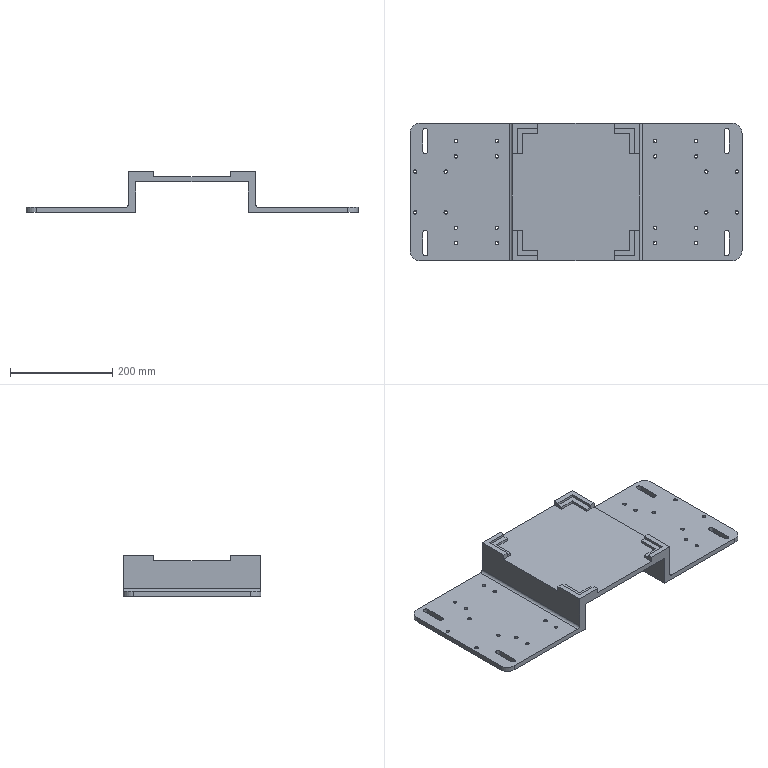Component | NX | MACHINING_PLATFORM | 1 solid | 140 faces | volume 2270417 mm3 | plane 54 | cone 48 | cylinder 38 | commonest cylinder face diameters 6 x24 10 x10 40 x4